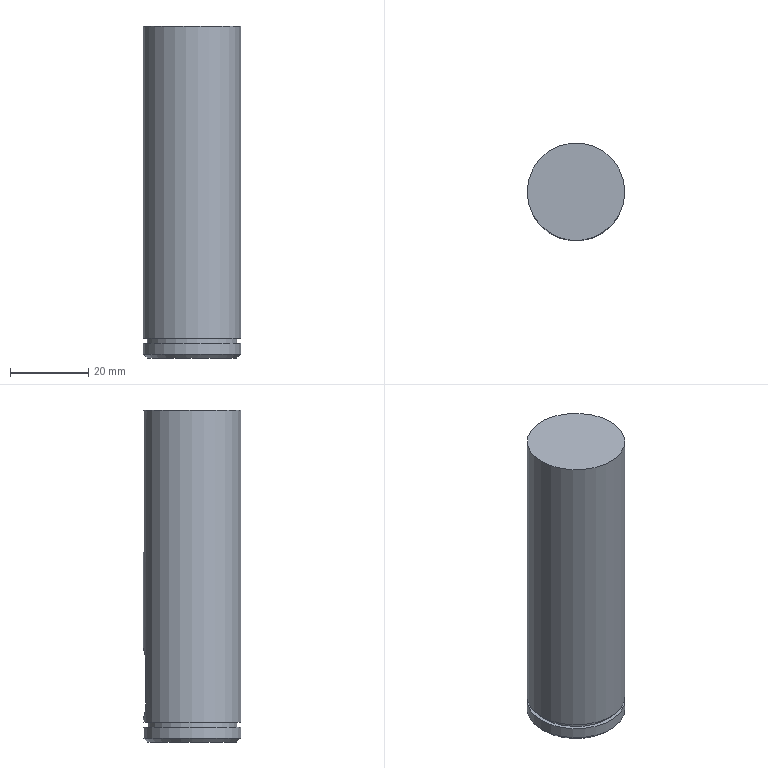Component | NX | MOTOR_SHAFT | 1 solid | 13 faces | box 25 x 25 x 85 mm | volume 41100 mm3 | plane 7 | cylinder 5 | cone 1 | commonest cylinder face diameters 25 x2 8 x2 23 x1
STEP:
#1=CARTESIAN_POINT('',(0.,0.,0.));
#2=DIRECTION('',(0.,0.,1.));
#3=DIRECTION('',(1.,0.,0.));
#4=AXIS2_PLACEMENT_3D('',#1,#2,#3);
#5=CARTESIAN_POINT('',(-610.675,308.181,-704.));
#6=VERTEX_POINT('',#5);
#7=CARTESIAN_POINT('',(-585.675,308.181,-704.));
#8=VERTEX_POINT('',#7);
#9=CARTESIAN_POINT('',(-598.175,308.181,-704.));
#10=DIRECTION('',(0.,0.,1.));
#11=DIRECTION('',(-1.,0.,0.));
#12=AXIS2_PLACEMENT_3D('',#9,#10,#11);
#13=CIRCLE('',#12,12.5);
#14=CARTESIAN_POINT('',(-598.175,308.181,-700.));
#15=DIRECTION('',(0.,0.,1.));
#16=DIRECTION('',(1.,0.,0.));
#17=AXIS2_PLACEMENT_3D('',#14,#15,#16);
#18=CYLINDRICAL_SURFACE('',#17,12.5);
#19=CARTESIAN_POINT('',(3.142,-4.));
#20=DIRECTION('',(1.,0.));
#21=VECTOR('',#20,1.);
#22=LINE('',#19,#21);
#23=(GEOMETRIC_REPRESENTATION_CONTEXT(2)PARAMETRIC_REPRESENTATION_CONTEXT()REPRESENTATION_CONTEXT('',''));
#24=DEFINITIONAL_REPRESENTATION('',(#22),#23);
#25=PCURVE('',#18,#24);
#26=CARTESIAN_POINT('',(-598.175,308.181,-704.));
#27=DIRECTION('',(0.,0.,1.));
#28=DIRECTION('',(1.,0.,0.));
#29=AXIS2_PLACEMENT_3D('',#26,#27,#28);
#30=CONICAL_SURFACE('',#29,12.5,0.7854);
#31=CARTESIAN_POINT('',(3.142,0.));
#32=DIRECTION('',(1.,0.));
#33=VECTOR('',#32,1.);
#34=LINE('',#31,#33);
#35=(GEOMETRIC_REPRESENTATION_CONTEXT(2)PARAMETRIC_REPRESENTATION_CONTEXT()REPRESENTATION_CONTEXT('',''));
#36=DEFINITIONAL_REPRESENTATION('',(#34),#35);
#37=PCURVE('',#30,#36);
#38=SURFACE_CURVE('',#13,(#25,#37),.PCURVE_S1.);
#39=EDGE_CURVE('',#6,#8,#38,.T.);
#40=ORIENTED_EDGE('',*,*,#39,.T.);
#41=CARTESIAN_POINT('',(-585.675,308.181,-701.2));
#42=VERTEX_POINT('',#41);
#43=CARTESIAN_POINT('',(-585.675,308.181,-704.));
#44=CARTESIAN_POINT('',(-585.675,308.181,-701.2));
#45=B_SPLINE_CURVE_WITH_KNOTS('',1,(#43,#44),.UNSPECIFIED.,.F.,.F.,(2,2),(-4.,-1.2),.PIECEWISE_BEZIER_KNOTS.);
#46=CARTESIAN_POINT('',(6.283,0.));
#47=DIRECTION('',(0.,1.));
#48=VECTOR('',#47,1.);
#49=LINE('',#46,#48);
#50=(GEOMETRIC_REPRESENTATION_CONTEXT(2)PARAMETRIC_REPRESENTATION_CONTEXT()REPRESENTATION_CONTEXT('',''));
#51=DEFINITIONAL_REPRESENTATION('',(#49),#50);
#52=PCURVE('',#18,#51);
#53=CARTESIAN_POINT('',(0.,0.));
#54=DIRECTION('',(0.,1.));
#55=VECTOR('',#54,1.);
#56=LINE('',#53,#55);
#57=(GEOMETRIC_REPRESENTATION_CONTEXT(2)PARAMETRIC_REPRESENTATION_CONTEXT()REPRESENTATION_CONTEXT('',''));
#58=DEFINITIONAL_REPRESENTATION('',(#56),#57);
#59=PCURVE('',#18,#58);
#60=SEAM_CURVE('',#45,(#52,#59),.PCURVE_S1.);
#61=EDGE_CURVE('',#8,#42,#60,.T.);
#62=ORIENTED_EDGE('',*,*,#61,.T.);
#63=CARTESIAN_POINT('',(-598.175,308.181,-701.2));
#64=DIRECTION('',(0.,0.,-1.));
#65=DIRECTION('',(1.,0.,0.));
#66=AXIS2_PLACEMENT_3D('',#63,#64,#65);
#67=CIRCLE('',#66,12.5);
#68=CARTESIAN_POINT('',(6.283,-1.2));
#69=DIRECTION('',(-1.,0.));
#70=VECTOR('',#69,1.);
#71=LINE('',#68,#70);
#72=(GEOMETRIC_REPRESENTATION_CONTEXT(2)PARAMETRIC_REPRESENTATION_CONTEXT()REPRESENTATION_CONTEXT('',''));
#73=DEFINITIONAL_REPRESENTATION('',(#71),#72);
#74=PCURVE('',#18,#73);
#75=CARTESIAN_POINT('',(-598.175,308.181,-701.2));
#76=DIRECTION('',(0.,0.,1.));
#77=DIRECTION('',(1.,0.,0.));
#78=AXIS2_PLACEMENT_3D('',#75,#76,#77);
#79=PLANE('',#78);
#80=CARTESIAN_POINT('',(12.5,0.));
#81=CARTESIAN_POINT('',(12.5,-21.651));
#82=CARTESIAN_POINT('',(-6.25,-10.825));
#83=CARTESIAN_POINT('',(-25.,-0.));
#84=CARTESIAN_POINT('',(-6.25,10.825));
#85=CARTESIAN_POINT('',(12.5,21.651));
#86=CARTESIAN_POINT('',(12.5,0.));
#87=(BOUNDED_CURVE()B_SPLINE_CURVE(2,(#80,#81,#82,#83,#84,#85,#86),.UNSPECIFIED.,.T.,.F.)B_SPLINE_CURVE_WITH_KNOTS((1,2,2,2,2,1),(-2.094,0.,2.094,4.189,6.283,8.378),.UNSPECIFIED.)CURVE()GEOMETRIC_REPRESENTATION_ITEM()RATIONAL_B_SPLINE_CURVE((1.,0.5,1.,0.5,1.,0.5,1.))REPRESENTATION_ITEM(''));
#88=(GEOMETRIC_REPRESENTATION_CONTEXT(2)PARAMETRIC_REPRESENTATION_CONTEXT()REPRESENTATION_CONTEXT('',''));
#89=DEFINITIONAL_REPRESENTATION('',(#87),#88);
#90=PCURVE('',#79,#89);
#91=SURFACE_CURVE('',#67,(#74,#90),.PCURVE_S1.);
#92=EDGE_CURVE('',#42,#42,#91,.T.);
#93=ORIENTED_EDGE('',*,*,#92,.T.);
#94=ORIENTED_EDGE('',*,*,#61,.F.);
#95=CARTESIAN_POINT('',(-598.175,308.181,-704.));
#96=DIRECTION('',(0.,0.,1.));
#97=DIRECTION('',(-1.,0.,0.));
#98=AXIS2_PLACEMENT_3D('',#95,#96,#97);
#99=CIRCLE('',#98,12.5);
#100=CARTESIAN_POINT('',(-3.142,-4.));
#101=DIRECTION('',(1.,0.));
#102=VECTOR('',#101,1.);
#103=LINE('',#100,#102);
#104=(GEOMETRIC_REPRESENTATION_CONTEXT(2)PARAMETRIC_REPRESENTATION_CONTEXT()REPRESENTATION_CONTEXT('',''));
#105=DEFINITIONAL_REPRESENTATION('',(#103),#104);
#106=PCURVE('',#18,#105);
#107=CARTESIAN_POINT('',(3.142,0.));
#108=DIRECTION('',(1.,0.));
#109=VECTOR('',#108,1.);
#110=LINE('',#107,#109);
#111=(GEOMETRIC_REPRESENTATION_CONTEXT(2)PARAMETRIC_REPRESENTATION_CONTEXT()REPRESENTATION_CONTEXT('',''));
#112=DEFINITIONAL_REPRESENTATION('',(#110),#111);
#113=PCURVE('',#30,#112);
#114=SURFACE_CURVE('',#99,(#106,#113),.PCURVE_S1.);
#115=EDGE_CURVE('',#8,#6,#114,.T.);
#116=ORIENTED_EDGE('',*,*,#115,.T.);
#117=EDGE_LOOP('',(#40,#62,#93,#94,#116));
#118=FACE_BOUND('',#117,.T.);
#119=ADVANCED_FACE('',(#118),#18,.T.);
#120=CARTESIAN_POINT('',(-609.675,308.181,-705.));
#121=VERTEX_POINT('',#120);
#122=CARTESIAN_POINT('',(-598.175,308.181,-705.));
#123=DIRECTION('',(0.,0.,-1.));
#124=DIRECTION('',(-1.,0.,0.));
#125=AXIS2_PLACEMENT_3D('',#122,#123,#124);
#126=CIRCLE('',#125,11.5);
#127=CARTESIAN_POINT('',(-598.175,308.181,-705.));
#128=DIRECTION('',(0.,0.,-1.));
#129=DIRECTION('',(-1.,0.,0.));
#130=AXIS2_PLACEMENT_3D('',#127,#128,#129);
#131=PLANE('',#130);
#132=CARTESIAN_POINT('',(0.,0.));
#133=DIRECTION('',(1.,0.));
#134=AXIS2_PLACEMENT_2D('',#132,#133);
#135=CIRCLE('',#134,11.5);
#136=(GEOMETRIC_REPRESENTATION_CONTEXT(2)PARAMETRIC_REPRESENTATION_CONTEXT()REPRESENTATION_CONTEXT('',''));
#137=DEFINITIONAL_REPRESENTATION('',(#135),#136);
#138=PCURVE('',#131,#137);
#139=CARTESIAN_POINT('',(9.425,-1.));
#140=DIRECTION('',(-1.,0.));
#141=VECTOR('',#140,1.);
#142=LINE('',#139,#141);
#143=(GEOMETRIC_REPRESENTATION_CONTEXT(2)PARAMETRIC_REPRESENTATION_CONTEXT()REPRESENTATION_CONTEXT('',''));
#144=DEFINITIONAL_REPRESENTATION('',(#142),#143);
#145=PCURVE('',#30,#144);
#146=SURFACE_CURVE('',#126,(#138,#145),.PCURVE_S1.);
#147=EDGE_CURVE('',#121,#121,#146,.T.);
#148=ORIENTED_EDGE('',*,*,#147,.T.);
#149=EDGE_LOOP('',(#148));
#150=FACE_BOUND('',#149,.T.);
#151=ADVANCED_FACE('',(#150),#131,.T.);
#152=ORIENTED_EDGE('',*,*,#147,.F.);
#153=CARTESIAN_POINT('',(-609.675,308.181,-705.));
#154=CARTESIAN_POINT('',(-610.675,308.181,-704.));
#155=B_SPLINE_CURVE_WITH_KNOTS('',1,(#153,#154),.UNSPECIFIED.,.F.,.F.,(2,2),(-1.414,0.),.PIECEWISE_BEZIER_KNOTS.);
#156=CARTESIAN_POINT('',(9.425,0.));
#157=DIRECTION('',(0.,1.));
#158=VECTOR('',#157,1.);
#159=LINE('',#156,#158);
#160=(GEOMETRIC_REPRESENTATION_CONTEXT(2)PARAMETRIC_REPRESENTATION_CONTEXT()REPRESENTATION_CONTEXT('',''));
#161=DEFINITIONAL_REPRESENTATION('',(#159),#160);
#162=PCURVE('',#30,#161);
#163=CARTESIAN_POINT('',(3.142,0.));
#164=DIRECTION('',(0.,1.));
#165=VECTOR('',#164,1.);
#166=LINE('',#163,#165);
#167=(GEOMETRIC_REPRESENTATION_CONTEXT(2)PARAMETRIC_REPRESENTATION_CONTEXT()REPRESENTATION_CONTEXT('',''));
#168=DEFINITIONAL_REPRESENTATION('',(#166),#167);
#169=PCURVE('',#30,#168);
#170=SEAM_CURVE('',#155,(#162,#169),.PCURVE_S1.);
#171=EDGE_CURVE('',#121,#6,#170,.T.);
#172=ORIENTED_EDGE('',*,*,#171,.T.);
#173=ORIENTED_EDGE('',*,*,#115,.F.);
#174=ORIENTED_EDGE('',*,*,#39,.F.);
#175=ORIENTED_EDGE('',*,*,#171,.F.);
#176=EDGE_LOOP('',(#152,#172,#173,#174,#175));
#177=FACE_BOUND('',#176,.T.);
#178=ADVANCED_FACE('',(#177),#30,.T.);
#179=CARTESIAN_POINT('',(-586.675,308.181,-700.));
#180=VERTEX_POINT('',#179);
#181=CARTESIAN_POINT('',(-598.175,308.181,-700.));
#182=DIRECTION('',(0.,0.,-1.));
#183=DIRECTION('',(1.,0.,0.));
#184=AXIS2_PLACEMENT_3D('',#181,#182,#183);
#185=CIRCLE('',#184,11.5);
#186=CARTESIAN_POINT('',(-598.175,308.181,-700.6));
#187=DIRECTION('',(0.,0.,1.));
#188=DIRECTION('',(1.,0.,0.));
#189=AXIS2_PLACEMENT_3D('',#186,#187,#188);
#190=CYLINDRICAL_SURFACE('',#189,11.5);
#191=CARTESIAN_POINT('',(6.283,0.6));
#192=DIRECTION('',(-1.,0.));
#193=VECTOR('',#192,1.);
#194=LINE('',#191,#193);
#195=(GEOMETRIC_REPRESENTATION_CONTEXT(2)PARAMETRIC_REPRESENTATION_CONTEXT()REPRESENTATION_CONTEXT('',''));
#196=DEFINITIONAL_REPRESENTATION('',(#194),#195);
#197=PCURVE('',#190,#196);
#198=CARTESIAN_POINT('',(-598.175,308.181,-700.));
#199=DIRECTION('',(0.,0.,1.));
#200=DIRECTION('',(1.,0.,0.));
#201=AXIS2_PLACEMENT_3D('',#198,#199,#200);
#202=PLANE('',#201);
#203=CARTESIAN_POINT('',(11.5,0.));
#204=CARTESIAN_POINT('',(11.5,-19.919));
#205=CARTESIAN_POINT('',(-5.75,-9.959));
#206=CARTESIAN_POINT('',(-23.,-0.));
#207=CARTESIAN_POINT('',(-5.75,9.959));
#208=CARTESIAN_POINT('',(11.5,19.919));
#209=CARTESIAN_POINT('',(11.5,0.));
#210=(BOUNDED_CURVE()B_SPLINE_CURVE(2,(#203,#204,#205,#206,#207,#208,#209),.UNSPECIFIED.,.T.,.F.)B_SPLINE_CURVE_WITH_KNOTS((1,2,2,2,2,1),(-2.094,0.,2.094,4.189,6.283,8.378),.UNSPECIFIED.)CURVE()GEOMETRIC_REPRESENTATION_ITEM()RATIONAL_B_SPLINE_CURVE((1.,0.5,1.,0.5,1.,0.5,1.))REPRESENTATION_ITEM(''));
#211=(GEOMETRIC_REPRESENTATION_CONTEXT(2)PARAMETRIC_REPRESENTATION_CONTEXT()REPRESENTATION_CONTEXT('',''));
#212=DEFINITIONAL_REPRESENTATION('',(#210),#211);
#213=PCURVE('',#202,#212);
#214=SURFACE_CURVE('',#185,(#197,#213),.PCURVE_S1.);
#215=EDGE_CURVE('',#180,#180,#214,.T.);
#216=ORIENTED_EDGE('',*,*,#215,.T.);
#217=CARTESIAN_POINT('',(-586.675,308.181,-701.2));
#218=VERTEX_POINT('',#217);
#219=CARTESIAN_POINT('',(-586.675,308.181,-701.2));
#220=CARTESIAN_POINT('',(-586.675,308.181,-700.));
#221=B_SPLINE_CURVE_WITH_KNOTS('',1,(#219,#220),.UNSPECIFIED.,.F.,.F.,(2,2),(-0.6,0.6),.PIECEWISE_BEZIER_KNOTS.);
#222=CARTESIAN_POINT('',(0.,0.));
#223=DIRECTION('',(0.,1.));
#224=VECTOR('',#223,1.);
#225=LINE('',#222,#224);
#226=(GEOMETRIC_REPRESENTATION_CONTEXT(2)PARAMETRIC_REPRESENTATION_CONTEXT()REPRESENTATION_CONTEXT('',''));
#227=DEFINITIONAL_REPRESENTATION('',(#225),#226);
#228=PCURVE('',#190,#227);
#229=CARTESIAN_POINT('',(6.283,0.));
#230=DIRECTION('',(0.,1.));
#231=VECTOR('',#230,1.);
#232=LINE('',#229,#231);
#233=(GEOMETRIC_REPRESENTATION_CONTEXT(2)PARAMETRIC_REPRESENTATION_CONTEXT()REPRESENTATION_CONTEXT('',''));
#234=DEFINITIONAL_REPRESENTATION('',(#232),#233);
#235=PCURVE('',#190,#234);
#236=SEAM_CURVE('',#221,(#228,#235),.PCURVE_S1.);
#237=EDGE_CURVE('',#218,#180,#236,.T.);
#238=ORIENTED_EDGE('',*,*,#237,.F.);
#239=CARTESIAN_POINT('',(-598.175,308.181,-701.2));
#240=DIRECTION('',(0.,0.,-1.));
#241=DIRECTION('',(1.,0.,0.));
#242=AXIS2_PLACEMENT_3D('',#239,#240,#241);
#243=CIRCLE('',#242,11.5);
#244=CARTESIAN_POINT('',(6.283,-0.6));
#245=DIRECTION('',(-1.,0.));
#246=VECTOR('',#245,1.);
#247=LINE('',#244,#246);
#248=(GEOMETRIC_REPRESENTATION_CONTEXT(2)PARAMETRIC_REPRESENTATION_CONTEXT()REPRESENTATION_CONTEXT('',''));
#249=DEFINITIONAL_REPRESENTATION('',(#247),#248);
#250=PCURVE('',#190,#249);
#251=CARTESIAN_POINT('',(11.5,0.));
#252=CARTESIAN_POINT('',(11.5,-19.919));
#253=CARTESIAN_POINT('',(-5.75,-9.959));
#254=CARTESIAN_POINT('',(-23.,-0.));
#255=CARTESIAN_POINT('',(-5.75,9.959));
#256=CARTESIAN_POINT('',(11.5,19.919));
#257=CARTESIAN_POINT('',(11.5,0.));
#258=(BOUNDED_CURVE()B_SPLINE_CURVE(2,(#251,#252,#253,#254,#255,#256,#257),.UNSPECIFIED.,.T.,.F.)B_SPLINE_CURVE_WITH_KNOTS((1,2,2,2,2,1),(-2.094,0.,2.094,4.189,6.283,8.378),.UNSPECIFIED.)CURVE()GEOMETRIC_REPRESENTATION_ITEM()RATIONAL_B_SPLINE_CURVE((1.,0.5,1.,0.5,1.,0.5,1.))REPRESENTATION_ITEM(''));
#259=(GEOMETRIC_REPRESENTATION_CONTEXT(2)PARAMETRIC_REPRESENTATION_CONTEXT()REPRESENTATION_CONTEXT('',''));
#260=DEFINITIONAL_REPRESENTATION('',(#258),#259);
#261=PCURVE('',#79,#260);
#262=SURFACE_CURVE('',#243,(#250,#261),.PCURVE_S1.);
#263=EDGE_CURVE('',#218,#218,#262,.T.);
#264=ORIENTED_EDGE('',*,*,#263,.F.);
#265=ORIENTED_EDGE('',*,*,#237,.T.);
#266=EDGE_LOOP('',(#216,#238,#264,#265));
#267=FACE_BOUND('',#266,.T.);
#268=ADVANCED_FACE('',(#267),#190,.T.);
#269=ORIENTED_EDGE('',*,*,#92,.F.);
#270=EDGE_LOOP('',(#269));
#271=FACE_BOUND('',#270,.T.);
#272=ORIENTED_EDGE('',*,*,#263,.T.);
#273=EDGE_LOOP('',(#272));
#274=FACE_BOUND('',#273,.T.);
#275=ADVANCED_FACE('',(#271,#274),#79,.T.);
#276=CARTESIAN_POINT('',(-585.675,308.181,-700.));
#277=VERTEX_POINT('',#276);
#278=CARTESIAN_POINT('',(-598.175,308.181,-700.));
#279=DIRECTION('',(0.,0.,-1.));
#280=DIRECTION('',(1.,0.,0.));
#281=AXIS2_PLACEMENT_3D('',#278,#279,#280);
#282=CIRCLE('',#281,12.5);
#283=CARTESIAN_POINT('',(12.5,0.));
#284=CARTESIAN_POINT('',(12.5,-21.651));
#285=CARTESIAN_POINT('',(-6.25,-10.825));
#286=CARTESIAN_POINT('',(-25.,-0.));
#287=CARTESIAN_POINT('',(-6.25,10.825));
#288=CARTESIAN_POINT('',(12.5,21.651));
#289=CARTESIAN_POINT('',(12.5,0.));
#290=(BOUNDED_CURVE()B_SPLINE_CURVE(2,(#283,#284,#285,#286,#287,#288,#289),.UNSPECIFIED.,.T.,.F.)B_SPLINE_CURVE_WITH_KNOTS((1,2,2,2,2,1),(-2.094,0.,2.094,4.189,6.283,8.378),.UNSPECIFIED.)CURVE()GEOMETRIC_REPRESENTATION_ITEM()RATIONAL_B_SPLINE_CURVE((1.,0.5,1.,0.5,1.,0.5,1.))REPRESENTATION_ITEM(''));
#291=(GEOMETRIC_REPRESENTATION_CONTEXT(2)PARAMETRIC_REPRESENTATION_CONTEXT()REPRESENTATION_CONTEXT('',''));
#292=DEFINITIONAL_REPRESENTATION('',(#290),#291);
#293=PCURVE('',#202,#292);
#294=CARTESIAN_POINT('',(-598.175,308.181,-700.));
#295=DIRECTION('',(0.,0.,1.));
#296=DIRECTION('',(1.,0.,0.));
#297=AXIS2_PLACEMENT_3D('',#294,#295,#296);
#298=CYLINDRICAL_SURFACE('',#297,12.5);
#299=CARTESIAN_POINT('',(6.283,0.));
#300=DIRECTION('',(-1.,0.));
#301=VECTOR('',#300,1.);
#302=LINE('',#299,#301);
#303=(GEOMETRIC_REPRESENTATION_CONTEXT(2)PARAMETRIC_REPRESENTATION_CONTEXT()REPRESENTATION_CONTEXT('',''));
#304=DEFINITIONAL_REPRESENTATION('',(#302),#303);
#305=PCURVE('',#298,#304);
#306=SURFACE_CURVE('',#282,(#293,#305),.PCURVE_S1.);
#307=EDGE_CURVE('',#277,#277,#306,.T.);
#308=ORIENTED_EDGE('',*,*,#307,.T.);
#309=EDGE_LOOP('',(#308));
#310=FACE_BOUND('',#309,.T.);
#311=ORIENTED_EDGE('',*,*,#215,.F.);
#312=EDGE_LOOP('',(#311));
#313=FACE_BOUND('',#312,.T.);
#314=ADVANCED_FACE('',(#310,#313),#202,.F.);
#315=CARTESIAN_POINT('',(-594.175,316.681,-695.));
#316=VERTEX_POINT('',#315);
#317=CARTESIAN_POINT('',(-594.175,316.681,-685.));
#318=VERTEX_POINT('',#317);
#319=CARTESIAN_POINT('',(-594.175,316.681,-681.));
#320=DIRECTION('',(0.,-0.,1.));
#321=VECTOR('',#320,1.);
#322=LINE('',#319,#321);
#323=CARTESIAN_POINT('',(-594.175,316.681,-681.));
#324=DIRECTION('',(0.,1.,0.));
#325=DIRECTION('',(0.,-0.,1.));
#326=AXIS2_PLACEMENT_3D('',#323,#324,#325);
#327=PLANE('',#326);
#328=CARTESIAN_POINT('',(0.,0.));
#329=DIRECTION('',(1.,0.));
#330=VECTOR('',#329,1.);
#331=LINE('',#328,#330);
#332=(GEOMETRIC_REPRESENTATION_CONTEXT(2)PARAMETRIC_REPRESENTATION_CONTEXT()REPRESENTATION_CONTEXT('',''));
#333=DEFINITIONAL_REPRESENTATION('',(#331),#332);
#334=PCURVE('',#327,#333);
#335=CARTESIAN_POINT('',(-594.175,308.181,-700.));
#336=DIRECTION('',(1.,0.,0.));
#337=DIRECTION('',(0.,0.,-1.));
#338=AXIS2_PLACEMENT_3D('',#335,#336,#337);
#339=PLANE('',#338);
#340=CARTESIAN_POINT('',(-19.,8.5));
#341=DIRECTION('',(-1.,-0.));
#342=VECTOR('',#341,1.);
#343=LINE('',#340,#342);
#344=(GEOMETRIC_REPRESENTATION_CONTEXT(2)PARAMETRIC_REPRESENTATION_CONTEXT()REPRESENTATION_CONTEXT('',''));
#345=DEFINITIONAL_REPRESENTATION('',(#343),#344);
#346=PCURVE('',#339,#345);
#347=SURFACE_CURVE('',#322,(#334,#346),.PCURVE_S1.);
#348=EDGE_CURVE('',#316,#318,#347,.T.);
#349=ORIENTED_EDGE('',*,*,#348,.F.);
#350=CARTESIAN_POINT('',(-602.175,316.681,-695.));
#351=VERTEX_POINT('',#350);
#352=CARTESIAN_POINT('',(-598.175,316.681,-695.));
#353=DIRECTION('',(0.,1.,0.));
#354=DIRECTION('',(0.,-0.,1.));
#355=AXIS2_PLACEMENT_3D('',#352,#353,#354);
#356=CIRCLE('',#355,4.);
#357=CARTESIAN_POINT('',(-14.,-4.));
#358=DIRECTION('',(1.,0.));
#359=AXIS2_PLACEMENT_2D('',#357,#358);
#360=CIRCLE('',#359,4.);
#361=(GEOMETRIC_REPRESENTATION_CONTEXT(2)PARAMETRIC_REPRESENTATION_CONTEXT()REPRESENTATION_CONTEXT('',''));
#362=DEFINITIONAL_REPRESENTATION('',(#360),#361);
#363=PCURVE('',#327,#362);
#364=CARTESIAN_POINT('',(-598.175,316.681,-695.));
#365=DIRECTION('',(0.,1.,0.));
#366=DIRECTION('',(0.,-0.,1.));
#367=AXIS2_PLACEMENT_3D('',#364,#365,#366);
#368=CYLINDRICAL_SURFACE('',#367,4.);
#369=CARTESIAN_POINT('',(0.,0.));
#370=DIRECTION('',(1.,0.));
#371=VECTOR('',#370,1.);
#372=LINE('',#369,#371);
#373=(GEOMETRIC_REPRESENTATION_CONTEXT(2)PARAMETRIC_REPRESENTATION_CONTEXT()REPRESENTATION_CONTEXT('',''));
#374=DEFINITIONAL_REPRESENTATION('',(#372),#373);
#375=PCURVE('',#368,#374);
#376=SURFACE_CURVE('',#356,(#363,#375),.PCURVE_S1.);
#377=EDGE_CURVE('',#316,#351,#376,.T.);
#378=ORIENTED_EDGE('',*,*,#377,.T.);
#379=CARTESIAN_POINT('',(-602.175,316.681,-685.));
#380=VERTEX_POINT('',#379);
#381=CARTESIAN_POINT('',(-602.175,316.681,-681.));
#382=DIRECTION('',(0.,-0.,1.));
#383=VECTOR('',#382,1.);
#384=LINE('',#381,#383);
#385=CARTESIAN_POINT('',(0.,-8.));
#386=DIRECTION('',(1.,0.));
#387=VECTOR('',#386,1.);
#388=LINE('',#385,#387);
#389=(GEOMETRIC_REPRESENTATION_CONTEXT(2)PARAMETRIC_REPRESENTATION_CONTEXT()REPRESENTATION_CONTEXT('',''));
#390=DEFINITIONAL_REPRESENTATION('',(#388),#389);
#391=PCURVE('',#327,#390);
#392=CARTESIAN_POINT('',(-602.175,308.181,-700.));
#393=DIRECTION('',(1.,0.,0.));
#394=DIRECTION('',(0.,0.,-1.));
#395=AXIS2_PLACEMENT_3D('',#392,#393,#394);
#396=PLANE('',#395);
#397=CARTESIAN_POINT('',(-19.,8.5));
#398=DIRECTION('',(-1.,-0.));
#399=VECTOR('',#398,1.);
#400=LINE('',#397,#399);
#401=(GEOMETRIC_REPRESENTATION_CONTEXT(2)PARAMETRIC_REPRESENTATION_CONTEXT()REPRESENTATION_CONTEXT('',''));
#402=DEFINITIONAL_REPRESENTATION('',(#400),#401);
#403=PCURVE('',#396,#402);
#404=SURFACE_CURVE('',#384,(#391,#403),.PCURVE_S1.);
#405=EDGE_CURVE('',#351,#380,#404,.T.);
#406=ORIENTED_EDGE('',*,*,#405,.T.);
#407=CARTESIAN_POINT('',(-598.175,316.681,-685.));
#408=DIRECTION('',(0.,1.,0.));
#409=DIRECTION('',(0.,-0.,1.));
#410=AXIS2_PLACEMENT_3D('',#407,#408,#409);
#411=CIRCLE('',#410,4.);
#412=CARTESIAN_POINT('',(-4.,-4.));
#413=DIRECTION('',(1.,0.));
#414=AXIS2_PLACEMENT_2D('',#412,#413);
#415=CIRCLE('',#414,4.);
#416=(GEOMETRIC_REPRESENTATION_CONTEXT(2)PARAMETRIC_REPRESENTATION_CONTEXT()REPRESENTATION_CONTEXT('',''));
#417=DEFINITIONAL_REPRESENTATION('',(#415),#416);
#418=PCURVE('',#327,#417);
#419=CARTESIAN_POINT('',(-598.175,308.181,-685.));
#420=DIRECTION('',(0.,1.,0.));
#421=DIRECTION('',(0.,0.,1.));
#422=AXIS2_PLACEMENT_3D('',#419,#420,#421);
#423=CYLINDRICAL_SURFACE('',#422,4.);
#424=CARTESIAN_POINT('',(-6.283,8.5));
#425=DIRECTION('',(1.,0.));
#426=VECTOR('',#425,1.);
#427=LINE('',#424,#426);
#428=(GEOMETRIC_REPRESENTATION_CONTEXT(2)PARAMETRIC_REPRESENTATION_CONTEXT()REPRESENTATION_CONTEXT('',''));
#429=DEFINITIONAL_REPRESENTATION('',(#427),#428);
#430=PCURVE('',#423,#429);
#431=SURFACE_CURVE('',#411,(#418,#430),.PCURVE_S1.);
#432=EDGE_CURVE('',#380,#318,#431,.T.);
#433=ORIENTED_EDGE('',*,*,#432,.T.);
#434=EDGE_LOOP('',(#349,#378,#406,#433));
#435=FACE_BOUND('',#434,.T.);
#436=ADVANCED_FACE('',(#435),#327,.T.);
#437=CARTESIAN_POINT('',(-585.675,308.181,-620.));
#438=VERTEX_POINT('',#437);
#439=CARTESIAN_POINT('',(-598.175,308.181,-620.));
#440=DIRECTION('',(0.,0.,-1.));
#441=DIRECTION('',(1.,0.,0.));
#442=AXIS2_PLACEMENT_3D('',#439,#440,#441);
#443=CIRCLE('',#442,12.5);
#444=CARTESIAN_POINT('',(-598.175,308.181,-620.));
#445=DIRECTION('',(0.,0.,1.));
#446=DIRECTION('',(1.,0.,0.));
#447=AXIS2_PLACEMENT_3D('',#444,#445,#446);
#448=PLANE('',#447);
#449=CARTESIAN_POINT('',(12.5,0.));
#450=CARTESIAN_POINT('',(12.5,-21.651));
#451=CARTESIAN_POINT('',(-6.25,-10.825));
#452=CARTESIAN_POINT('',(-25.,-0.));
#453=CARTESIAN_POINT('',(-6.25,10.825));
#454=CARTESIAN_POINT('',(12.5,21.651));
#455=CARTESIAN_POINT('',(12.5,0.));
#456=(BOUNDED_CURVE()B_SPLINE_CURVE(2,(#449,#450,#451,#452,#453,#454,#455),.UNSPECIFIED.,.T.,.F.)B_SPLINE_CURVE_WITH_KNOTS((1,2,2,2,2,1),(-2.094,0.,2.094,4.189,6.283,8.378),.UNSPECIFIED.)CURVE()GEOMETRIC_REPRESENTATION_ITEM()RATIONAL_B_SPLINE_CURVE((1.,0.5,1.,0.5,1.,0.5,1.))REPRESENTATION_ITEM(''));
#457=(GEOMETRIC_REPRESENTATION_CONTEXT(2)PARAMETRIC_REPRESENTATION_CONTEXT()REPRESENTATION_CONTEXT('',''));
#458=DEFINITIONAL_REPRESENTATION('',(#456),#457);
#459=PCURVE('',#448,#458);
#460=CARTESIAN_POINT('',(6.283,80.));
#461=DIRECTION('',(-1.,0.));
#462=VECTOR('',#461,1.);
#463=LINE('',#460,#462);
#464=(GEOMETRIC_REPRESENTATION_CONTEXT(2)PARAMETRIC_REPRESENTATION_CONTEXT()REPRESENTATION_CONTEXT('',''));
#465=DEFINITIONAL_REPRESENTATION('',(#463),#464);
#466=PCURVE('',#298,#465);
#467=SURFACE_CURVE('',#443,(#459,#466),.PCURVE_S1.);
#468=EDGE_CURVE('',#438,#438,#467,.T.);
#469=ORIENTED_EDGE('',*,*,#468,.F.);
#470=EDGE_LOOP('',(#469));
#471=FACE_BOUND('',#470,.T.);
#472=ADVANCED_FACE('',(#471),#448,.T.);
#473=CARTESIAN_POINT('',(-602.175,320.024,-695.));
#474=VERTEX_POINT('',#473);
#475=CARTESIAN_POINT('',(-602.175,320.024,-695.));
#476=DIRECTION('',(0.,1.,0.));
#477=VECTOR('',#476,1.);
#478=LINE('',#475,#477);
#479=CARTESIAN_POINT('',(4.712,3.343));
#480=DIRECTION('',(0.,1.));
#481=VECTOR('',#480,1.);
#482=LINE('',#479,#481);
#483=(GEOMETRIC_REPRESENTATION_CONTEXT(2)PARAMETRIC_REPRESENTATION_CONTEXT()REPRESENTATION_CONTEXT('',''));
#484=DEFINITIONAL_REPRESENTATION('',(#482),#483);
#485=PCURVE('',#368,#484);
#486=CARTESIAN_POINT('',(-5.,11.843));
#487=DIRECTION('',(-0.,1.));
#488=VECTOR('',#487,1.);
#489=LINE('',#486,#488);
#490=(GEOMETRIC_REPRESENTATION_CONTEXT(2)PARAMETRIC_REPRESENTATION_CONTEXT()REPRESENTATION_CONTEXT('',''));
#491=DEFINITIONAL_REPRESENTATION('',(#489),#490);
#492=PCURVE('',#396,#491);
#493=SURFACE_CURVE('',#478,(#485,#492),.PCURVE_S1.);
#494=EDGE_CURVE('',#351,#474,#493,.T.);
#495=ORIENTED_EDGE('',*,*,#494,.T.);
#496=CARTESIAN_POINT('',(-594.175,320.024,-695.));
#497=VERTEX_POINT('',#496);
#498=CARTESIAN_POINT('',(-602.175,320.024,-695.));
#499=CARTESIAN_POINT('',(-602.175,320.024,-695.435));
#500=CARTESIAN_POINT('',(-602.102,320.049,-695.875));
#501=CARTESIAN_POINT('',(-601.963,320.094,-696.285));
#502=CARTESIAN_POINT('',(-601.824,320.138,-696.694));
#503=CARTESIAN_POINT('',(-601.617,320.201,-697.083));
#504=CARTESIAN_POINT('',(-601.357,320.27,-697.424));
#505=CARTESIAN_POINT('',(-601.088,320.34,-697.777));
#506=CARTESIAN_POINT('',(-600.757,320.418,-698.087));
#507=CARTESIAN_POINT('',(-600.388,320.484,-698.332));
#508=CARTESIAN_POINT('',(-600.01,320.552,-698.583));
#509=CARTESIAN_POINT('',(-599.58,320.61,-698.773));
#510=CARTESIAN_POINT('',(-599.136,320.644,-698.883));
#511=CARTESIAN_POINT('',(-598.823,320.668,-698.96));
#512=CARTESIAN_POINT('',(-598.498,320.681,-699.));
#513=CARTESIAN_POINT('',(-598.175,320.681,-699.));
#514=CARTESIAN_POINT('',(-597.74,320.681,-699.));
#515=CARTESIAN_POINT('',(-597.299,320.657,-698.927));
#516=CARTESIAN_POINT('',(-596.888,320.615,-698.787));
#517=CARTESIAN_POINT('',(-596.478,320.573,-698.648));
#518=CARTESIAN_POINT('',(-596.088,320.511,-698.439));
#519=CARTESIAN_POINT('',(-595.747,320.443,-698.179));
#520=CARTESIAN_POINT('',(-595.396,320.374,-697.91));
#521=CARTESIAN_POINT('',(-595.086,320.296,-697.579));
#522=CARTESIAN_POINT('',(-594.842,320.229,-697.21));
#523=CARTESIAN_POINT('',(-594.591,320.159,-696.832));
#524=CARTESIAN_POINT('',(-594.402,320.099,-696.403));
#525=CARTESIAN_POINT('',(-594.292,320.063,-695.959));
#526=CARTESIAN_POINT('',(-594.215,320.038,-695.647));
#527=CARTESIAN_POINT('',(-594.175,320.024,-695.322));
#528=CARTESIAN_POINT('',(-594.175,320.024,-695.));
#529=B_SPLINE_CURVE_WITH_KNOTS('',3,(#498,#499,#500,#501,#502,#503,#504,#505,#506,#507,#508,#509,#510,#511,#512,#513,#514,#515,#516,#517,#518,#519,#520,#521,#522,#523,#524,#525,#526,#527,#528),.UNSPECIFIED.,.F.,.F.,(4,3,3,3,3,3,3,3,3,3,4),(0.,0.1037,0.2071,0.314,0.4235,0.5,0.6038,0.7074,0.8141,0.9237,1.),.UNSPECIFIED.);
#530=CARTESIAN_POINT('',(4.712,3.343));
#531=CARTESIAN_POINT('',(4.689,3.343));
#532=CARTESIAN_POINT('',(4.641,3.345));
#533=CARTESIAN_POINT('',(4.569,3.356));
#534=CARTESIAN_POINT('',(4.497,3.373));
#535=CARTESIAN_POINT('',(4.425,3.396));
#536=CARTESIAN_POINT('',(4.354,3.425));
#537=CARTESIAN_POINT('',(4.283,3.459));
#538=CARTESIAN_POINT('',(4.211,3.497));
#539=CARTESIAN_POINT('',(4.14,3.539));
#540=CARTESIAN_POINT('',(4.069,3.583));
#541=CARTESIAN_POINT('',(3.999,3.629));
#542=CARTESIAN_POINT('',(3.928,3.675));
#543=CARTESIAN_POINT('',(3.856,3.722));
#544=CARTESIAN_POINT('',(3.785,3.768));
#545=CARTESIAN_POINT('',(3.715,3.811));
#546=CARTESIAN_POINT('',(3.644,3.851));
#547=CARTESIAN_POINT('',(3.572,3.888));
#548=CARTESIAN_POINT('',(3.501,3.921));
#549=CARTESIAN_POINT('',(3.429,3.949));
#550=CARTESIAN_POINT('',(3.358,3.971));
#551=CARTESIAN_POINT('',(3.286,3.988));
#552=CARTESIAN_POINT('',(3.214,3.998));
#553=CARTESIAN_POINT('',(3.141,4.001));
#554=CARTESIAN_POINT('',(3.07,3.998));
#555=CARTESIAN_POINT('',(2.998,3.988));
#556=CARTESIAN_POINT('',(2.926,3.972));
#557=CARTESIAN_POINT('',(2.854,3.949));
#558=CARTESIAN_POINT('',(2.783,3.922));
#559=CARTESIAN_POINT('',(2.712,3.889));
#560=CARTESIAN_POINT('',(2.64,3.852));
#561=CARTESIAN_POINT('',(2.569,3.811));
#562=CARTESIAN_POINT('',(2.498,3.768));
#563=CARTESIAN_POINT('',(2.428,3.723));
#564=CARTESIAN_POINT('',(2.357,3.676));
#565=CARTESIAN_POINT('',(2.285,3.629));
#566=CARTESIAN_POINT('',(2.214,3.583));
#567=CARTESIAN_POINT('',(2.144,3.539));
#568=CARTESIAN_POINT('',(2.073,3.498));
#569=CARTESIAN_POINT('',(2.001,3.459));
#570=CARTESIAN_POINT('',(1.93,3.425));
#571=CARTESIAN_POINT('',(1.859,3.396));
#572=CARTESIAN_POINT('',(1.787,3.373));
#573=CARTESIAN_POINT('',(1.715,3.356));
#574=CARTESIAN_POINT('',(1.643,3.345));
#575=CARTESIAN_POINT('',(1.595,3.343));
#576=CARTESIAN_POINT('',(1.571,3.343));
#577=B_SPLINE_CURVE_WITH_KNOTS('',3,(#530,#531,#532,#533,#534,#535,#536,#537,#538,#539,#540,#541,#542,#543,#544,#545,#546,#547,#548,#549,#550,#551,#552,#553,#554,#555,#556,#557,#558,#559,#560,#561,#562,#563,#564,#565,#566,#567,#568,#569,#570,#571,#572,#573,#574,#575,#576),.UNSPECIFIED.,.F.,.F.,(4,1,1,1,1,1,1,1,1,1,1,1,1,1,1,1,1,1,1,1,1,1,1,1,1,1,1,1,1,1,1,1,1,1,1,1,1,1,1,1,1,1,1,1,4),(0.,0.02273,0.04545,0.06818,0.09091,0.1136,0.1364,0.1591,0.1818,0.2045,0.2273,0.25,0.2727,0.2955,0.3182,0.3409,0.3636,0.3864,0.4091,0.4318,0.4545,0.4773,0.5,0.5227,0.5455,0.5682,0.5909,0.6136,0.6364,0.6591,0.6818,0.7045,0.7273,0.75,0.7727,0.7955,0.8182,0.8409,0.8636,0.8864,0.9091,0.9318,0.9545,0.9773,1.),.QUASI_UNIFORM_KNOTS.);
#578=(GEOMETRIC_REPRESENTATION_CONTEXT(2)PARAMETRIC_REPRESENTATION_CONTEXT()REPRESENTATION_CONTEXT('',''));
#579=DEFINITIONAL_REPRESENTATION('',(#577),#578);
#580=PCURVE('',#368,#579);
#581=CARTESIAN_POINT('',(1.897,5.));
#582=CARTESIAN_POINT('',(1.897,4.905));
#583=CARTESIAN_POINT('',(1.896,4.714));
#584=CARTESIAN_POINT('',(1.893,4.427));
#585=CARTESIAN_POINT('',(1.889,4.144));
#586=CARTESIAN_POINT('',(1.883,3.866));
#587=CARTESIAN_POINT('',(1.875,3.596));
#588=CARTESIAN_POINT('',(1.866,3.333));
#589=CARTESIAN_POINT('',(1.856,3.077));
#590=CARTESIAN_POINT('',(1.843,2.832));
#591=CARTESIAN_POINT('',(1.83,2.599));
#592=CARTESIAN_POINT('',(1.815,2.379));
#593=CARTESIAN_POINT('',(1.799,2.171));
#594=CARTESIAN_POINT('',(1.782,1.977));
#595=CARTESIAN_POINT('',(1.764,1.798));
#596=CARTESIAN_POINT('',(1.745,1.636));
#597=CARTESIAN_POINT('',(1.726,1.491));
#598=CARTESIAN_POINT('',(1.705,1.363));
#599=CARTESIAN_POINT('',(1.684,1.253));
#600=CARTESIAN_POINT('',(1.662,1.161));
#601=CARTESIAN_POINT('',(1.64,1.09));
#602=CARTESIAN_POINT('',(1.617,1.038));
#603=CARTESIAN_POINT('',(1.594,1.007));
#604=CARTESIAN_POINT('',(1.571,0.9965));
#605=CARTESIAN_POINT('',(1.548,1.007));
#606=CARTESIAN_POINT('',(1.525,1.038));
#607=CARTESIAN_POINT('',(1.502,1.09));
#608=CARTESIAN_POINT('',(1.48,1.161));
#609=CARTESIAN_POINT('',(1.458,1.251));
#610=CARTESIAN_POINT('',(1.437,1.361));
#611=CARTESIAN_POINT('',(1.416,1.489));
#612=CARTESIAN_POINT('',(1.396,1.635));
#613=CARTESIAN_POINT('',(1.377,1.797));
#614=CARTESIAN_POINT('',(1.359,1.975));
#615=CARTESIAN_POINT('',(1.342,2.169));
#616=CARTESIAN_POINT('',(1.326,2.377));
#617=CARTESIAN_POINT('',(1.312,2.598));
#618=CARTESIAN_POINT('',(1.298,2.83));
#619=CARTESIAN_POINT('',(1.286,3.074));
#620=CARTESIAN_POINT('',(1.276,3.329));
#621=CARTESIAN_POINT('',(1.266,3.593));
#622=CARTESIAN_POINT('',(1.259,3.864));
#623=CARTESIAN_POINT('',(1.253,4.14));
#624=CARTESIAN_POINT('',(1.248,4.424));
#625=CARTESIAN_POINT('',(1.246,4.712));
#626=CARTESIAN_POINT('',(1.245,4.904));
#627=CARTESIAN_POINT('',(1.245,5.));
#628=B_SPLINE_CURVE_WITH_KNOTS('',3,(#581,#582,#583,#584,#585,#586,#587,#588,#589,#590,#591,#592,#593,#594,#595,#596,#597,#598,#599,#600,#601,#602,#603,#604,#605,#606,#607,#608,#609,#610,#611,#612,#613,#614,#615,#616,#617,#618,#619,#620,#621,#622,#623,#624,#625,#626,#627),.UNSPECIFIED.,.F.,.F.,(4,1,1,1,1,1,1,1,1,1,1,1,1,1,1,1,1,1,1,1,1,1,1,1,1,1,1,1,1,1,1,1,1,1,1,1,1,1,1,1,1,1,1,1,4),(0.,0.02273,0.04545,0.06818,0.09091,0.1136,0.1364,0.1591,0.1818,0.2045,0.2273,0.25,0.2727,0.2955,0.3182,0.3409,0.3636,0.3864,0.4091,0.4318,0.4545,0.4773,0.5,0.5227,0.5455,0.5682,0.5909,0.6136,0.6364,0.6591,0.6818,0.7045,0.7273,0.75,0.7727,0.7955,0.8182,0.8409,0.8636,0.8864,0.9091,0.9318,0.9545,0.9773,1.),.QUASI_UNIFORM_KNOTS.);
#629=(GEOMETRIC_REPRESENTATION_CONTEXT(2)PARAMETRIC_REPRESENTATION_CONTEXT()REPRESENTATION_CONTEXT('',''));
#630=DEFINITIONAL_REPRESENTATION('',(#628),#629);
#631=PCURVE('',#298,#630);
#632=SURFACE_CURVE('',#529,(#580,#631),.PCURVE_S1.);
#633=EDGE_CURVE('',#474,#497,#632,.T.);
#634=ORIENTED_EDGE('',*,*,#633,.T.);
#635=CARTESIAN_POINT('',(-594.175,308.181,-695.));
#636=DIRECTION('',(0.,-1.,-0.));
#637=VECTOR('',#636,1.);
#638=LINE('',#635,#637);
#639=CARTESIAN_POINT('',(1.571,-8.5));
#640=DIRECTION('',(0.,-1.));
#641=VECTOR('',#640,1.);
#642=LINE('',#639,#641);
#643=(GEOMETRIC_REPRESENTATION_CONTEXT(2)PARAMETRIC_REPRESENTATION_CONTEXT()REPRESENTATION_CONTEXT('',''));
#644=DEFINITIONAL_REPRESENTATION('',(#642),#643);
#645=PCURVE('',#368,#644);
#646=CARTESIAN_POINT('',(-5.,0.));
#647=DIRECTION('',(0.,-1.));
#648=VECTOR('',#647,1.);
#649=LINE('',#646,#648);
#650=(GEOMETRIC_REPRESENTATION_CONTEXT(2)PARAMETRIC_REPRESENTATION_CONTEXT()REPRESENTATION_CONTEXT('',''));
#651=DEFINITIONAL_REPRESENTATION('',(#649),#650);
#652=PCURVE('',#339,#651);
#653=SURFACE_CURVE('',#638,(#645,#652),.PCURVE_S1.);
#654=EDGE_CURVE('',#497,#316,#653,.T.);
#655=ORIENTED_EDGE('',*,*,#654,.T.);
#656=ORIENTED_EDGE('',*,*,#377,.T.);
#657=EDGE_LOOP('',(#495,#634,#655,#656));
#658=FACE_BOUND('',#657,.F.);
#659=ADVANCED_FACE('',(#658),#368,.F.);
#660=ORIENTED_EDGE('',*,*,#405,.F.);
#661=ORIENTED_EDGE('',*,*,#494,.T.);
#662=CARTESIAN_POINT('',(-602.175,320.024,-685.));
#663=VERTEX_POINT('',#662);
#664=CARTESIAN_POINT('',(-602.175,320.024,-700.));
#665=DIRECTION('',(0.,0.,-1.));
#666=VECTOR('',#665,1.);
#667=LINE('',#664,#666);
#668=CARTESIAN_POINT('',(0.,11.843));
#669=DIRECTION('',(1.,0.));
#670=VECTOR('',#669,1.);
#671=LINE('',#668,#670);
#672=(GEOMETRIC_REPRESENTATION_CONTEXT(2)PARAMETRIC_REPRESENTATION_CONTEXT()REPRESENTATION_CONTEXT('',''));
#673=DEFINITIONAL_REPRESENTATION('',(#671),#672);
#674=PCURVE('',#396,#673);
#675=CARTESIAN_POINT('',(1.897,0.));
#676=DIRECTION('',(0.,-1.));
#677=VECTOR('',#676,1.);
#678=LINE('',#675,#677);
#679=(GEOMETRIC_REPRESENTATION_CONTEXT(2)PARAMETRIC_REPRESENTATION_CONTEXT()REPRESENTATION_CONTEXT('',''));
#680=DEFINITIONAL_REPRESENTATION('',(#678),#679);
#681=PCURVE('',#298,#680);
#682=SURFACE_CURVE('',#667,(#674,#681),.PCURVE_S1.);
#683=EDGE_CURVE('',#663,#474,#682,.T.);
#684=ORIENTED_EDGE('',*,*,#683,.F.);
#685=CARTESIAN_POINT('',(-602.175,316.681,-685.));
#686=DIRECTION('',(0.,-1.,0.));
#687=VECTOR('',#686,1.);
#688=LINE('',#685,#687);
#689=CARTESIAN_POINT('',(-15.,8.5));
#690=DIRECTION('',(0.,-1.));
#691=VECTOR('',#690,1.);
#692=LINE('',#689,#691);
#693=(GEOMETRIC_REPRESENTATION_CONTEXT(2)PARAMETRIC_REPRESENTATION_CONTEXT()REPRESENTATION_CONTEXT('',''));
#694=DEFINITIONAL_REPRESENTATION('',(#692),#693);
#695=PCURVE('',#396,#694);
#696=CARTESIAN_POINT('',(-1.571,8.5));
#697=DIRECTION('',(0.,-1.));
#698=VECTOR('',#697,1.);
#699=LINE('',#696,#698);
#700=(GEOMETRIC_REPRESENTATION_CONTEXT(2)PARAMETRIC_REPRESENTATION_CONTEXT()REPRESENTATION_CONTEXT('',''));
#701=DEFINITIONAL_REPRESENTATION('',(#699),#700);
#702=PCURVE('',#423,#701);
#703=SURFACE_CURVE('',#688,(#695,#702),.PCURVE_S1.);
#704=EDGE_CURVE('',#663,#380,#703,.T.);
#705=ORIENTED_EDGE('',*,*,#704,.T.);
#706=EDGE_LOOP('',(#660,#661,#684,#705));
#707=FACE_BOUND('',#706,.T.);
#708=ADVANCED_FACE('',(#707),#396,.T.);
#709=CARTESIAN_POINT('',(-594.175,320.024,-685.));
#710=VERTEX_POINT('',#709);
#711=CARTESIAN_POINT('',(-594.175,320.024,-685.));
#712=CARTESIAN_POINT('',(-594.175,320.024,-684.565));
#713=CARTESIAN_POINT('',(-594.248,320.049,-684.125));
#714=CARTESIAN_POINT('',(-594.387,320.094,-683.715));
#715=CARTESIAN_POINT('',(-594.526,320.138,-683.306));
#716=CARTESIAN_POINT('',(-594.734,320.201,-682.917));
#717=CARTESIAN_POINT('',(-594.994,320.27,-682.576));
#718=CARTESIAN_POINT('',(-595.262,320.34,-682.223));
#719=CARTESIAN_POINT('',(-595.593,320.418,-681.913));
#720=CARTESIAN_POINT('',(-595.963,320.484,-681.668));
#721=CARTESIAN_POINT('',(-596.341,320.552,-681.417));
#722=CARTESIAN_POINT('',(-596.77,320.61,-681.227));
#723=CARTESIAN_POINT('',(-597.215,320.644,-681.117));
#724=CARTESIAN_POINT('',(-597.527,320.668,-681.04));
#725=CARTESIAN_POINT('',(-597.852,320.681,-681.));
#726=CARTESIAN_POINT('',(-598.175,320.681,-681.));
#727=CARTESIAN_POINT('',(-598.611,320.681,-681.));
#728=CARTESIAN_POINT('',(-599.052,320.657,-681.073));
#729=CARTESIAN_POINT('',(-599.462,320.615,-681.213));
#730=CARTESIAN_POINT('',(-599.872,320.573,-681.352));
#731=CARTESIAN_POINT('',(-600.262,320.511,-681.561));
#732=CARTESIAN_POINT('',(-600.604,320.443,-681.821));
#733=CARTESIAN_POINT('',(-600.955,320.374,-682.09));
#734=CARTESIAN_POINT('',(-601.265,320.296,-682.421));
#735=CARTESIAN_POINT('',(-601.509,320.229,-682.79));
#736=CARTESIAN_POINT('',(-601.76,320.159,-683.168));
#737=CARTESIAN_POINT('',(-601.949,320.099,-683.597));
#738=CARTESIAN_POINT('',(-602.059,320.063,-684.041));
#739=CARTESIAN_POINT('',(-602.136,320.038,-684.353));
#740=CARTESIAN_POINT('',(-602.175,320.024,-684.678));
#741=CARTESIAN_POINT('',(-602.175,320.024,-685.));
#742=B_SPLINE_CURVE_WITH_KNOTS('',3,(#711,#712,#713,#714,#715,#716,#717,#718,#719,#720,#721,#722,#723,#724,#725,#726,#727,#728,#729,#730,#731,#732,#733,#734,#735,#736,#737,#738,#739,#740,#741),.UNSPECIFIED.,.F.,.F.,(4,3,3,3,3,3,3,3,3,3,4),(0.,0.1037,0.2071,0.314,0.4235,0.5,0.6038,0.7074,0.8141,0.9237,1.),.UNSPECIFIED.);
#743=CARTESIAN_POINT('',(1.571,11.843));
#744=CARTESIAN_POINT('',(1.547,11.843));
#745=CARTESIAN_POINT('',(1.499,11.845));
#746=CARTESIAN_POINT('',(1.427,11.856));
#747=CARTESIAN_POINT('',(1.355,11.873));
#748=CARTESIAN_POINT('',(1.284,11.896));
#749=CARTESIAN_POINT('',(1.213,11.925));
#750=CARTESIAN_POINT('',(1.141,11.959));
#751=CARTESIAN_POINT('',(1.07,11.997));
#752=CARTESIAN_POINT('',(0.9985,12.039));
#753=CARTESIAN_POINT('',(0.9276,12.083));
#754=CARTESIAN_POINT('',(0.857,12.129));
#755=CARTESIAN_POINT('',(0.7859,12.175));
#756=CARTESIAN_POINT('',(0.7149,12.222));
#757=CARTESIAN_POINT('',(0.6438,12.268));
#758=CARTESIAN_POINT('',(0.5731,12.311));
#759=CARTESIAN_POINT('',(0.5022,12.351));
#760=CARTESIAN_POINT('',(0.4308,12.388));
#761=CARTESIAN_POINT('',(0.3593,12.421));
#762=CARTESIAN_POINT('',(0.2878,12.449));
#763=CARTESIAN_POINT('',(0.2165,12.471));
#764=CARTESIAN_POINT('',(0.1443,12.488));
#765=CARTESIAN_POINT('',(0.07209,12.498));
#766=CARTESIAN_POINT('',(-0.0001412,12.501));
#767=CARTESIAN_POINT('',(-0.07158,12.498));
#768=CARTESIAN_POINT('',(-0.1436,12.488));
#769=CARTESIAN_POINT('',(-0.2155,12.472));
#770=CARTESIAN_POINT('',(-0.2872,12.449));
#771=CARTESIAN_POINT('',(-0.3583,12.422));
#772=CARTESIAN_POINT('',(-0.4297,12.389));
#773=CARTESIAN_POINT('',(-0.5012,12.352));
#774=CARTESIAN_POINT('',(-0.5725,12.311));
#775=CARTESIAN_POINT('',(-0.6434,12.268));
#776=CARTESIAN_POINT('',(-0.7141,12.223));
#777=CARTESIAN_POINT('',(-0.7851,12.176));
#778=CARTESIAN_POINT('',(-0.8562,12.129));
#779=CARTESIAN_POINT('',(-0.9272,12.083));
#780=CARTESIAN_POINT('',(-0.9979,12.039));
#781=CARTESIAN_POINT('',(-1.069,11.998));
#782=CARTESIAN_POINT('',(-1.14,11.959));
#783=CARTESIAN_POINT('',(-1.212,11.925));
#784=CARTESIAN_POINT('',(-1.283,11.896));
#785=CARTESIAN_POINT('',(-1.354,11.873));
#786=CARTESIAN_POINT('',(-1.427,11.856));
#787=CARTESIAN_POINT('',(-1.499,11.845));
#788=CARTESIAN_POINT('',(-1.547,11.843));
#789=CARTESIAN_POINT('',(-1.571,11.843));
#790=B_SPLINE_CURVE_WITH_KNOTS('',3,(#743,#744,#745,#746,#747,#748,#749,#750,#751,#752,#753,#754,#755,#756,#757,#758,#759,#760,#761,#762,#763,#764,#765,#766,#767,#768,#769,#770,#771,#772,#773,#774,#775,#776,#777,#778,#779,#780,#781,#782,#783,#784,#785,#786,#787,#788,#789),.UNSPECIFIED.,.F.,.F.,(4,1,1,1,1,1,1,1,1,1,1,1,1,1,1,1,1,1,1,1,1,1,1,1,1,1,1,1,1,1,1,1,1,1,1,1,1,1,1,1,1,1,1,1,4),(0.,0.02273,0.04545,0.06818,0.09091,0.1136,0.1364,0.1591,0.1818,0.2045,0.2273,0.25,0.2727,0.2955,0.3182,0.3409,0.3636,0.3864,0.4091,0.4318,0.4545,0.4773,0.5,0.5227,0.5455,0.5682,0.5909,0.6136,0.6364,0.6591,0.6818,0.7045,0.7273,0.75,0.7727,0.7955,0.8182,0.8409,0.8636,0.8864,0.9091,0.9318,0.9545,0.9773,1.),.QUASI_UNIFORM_KNOTS.);
#791=(GEOMETRIC_REPRESENTATION_CONTEXT(2)PARAMETRIC_REPRESENTATION_CONTEXT()REPRESENTATION_CONTEXT('',''));
#792=DEFINITIONAL_REPRESENTATION('',(#790),#791);
#793=PCURVE('',#423,#792);
#794=CARTESIAN_POINT('',(1.245,15.));
#795=CARTESIAN_POINT('',(1.245,15.095));
#796=CARTESIAN_POINT('',(1.246,15.286));
#797=CARTESIAN_POINT('',(1.248,15.573));
#798=CARTESIAN_POINT('',(1.253,15.856));
#799=CARTESIAN_POINT('',(1.259,16.134));
#800=CARTESIAN_POINT('',(1.266,16.404));
#801=CARTESIAN_POINT('',(1.275,16.667));
#802=CARTESIAN_POINT('',(1.286,16.923));
#803=CARTESIAN_POINT('',(1.298,17.168));
#804=CARTESIAN_POINT('',(1.312,17.401));
#805=CARTESIAN_POINT('',(1.326,17.621));
#806=CARTESIAN_POINT('',(1.342,17.829));
#807=CARTESIAN_POINT('',(1.359,18.023));
#808=CARTESIAN_POINT('',(1.377,18.202));
#809=CARTESIAN_POINT('',(1.396,18.364));
#810=CARTESIAN_POINT('',(1.416,18.509));
#811=CARTESIAN_POINT('',(1.437,18.637));
#812=CARTESIAN_POINT('',(1.458,18.747));
#813=CARTESIAN_POINT('',(1.48,18.839));
#814=CARTESIAN_POINT('',(1.502,18.91));
#815=CARTESIAN_POINT('',(1.525,18.962));
#816=CARTESIAN_POINT('',(1.548,18.993));
#817=CARTESIAN_POINT('',(1.571,19.004));
#818=CARTESIAN_POINT('',(1.594,18.993));
#819=CARTESIAN_POINT('',(1.617,18.962));
#820=CARTESIAN_POINT('',(1.639,18.91));
#821=CARTESIAN_POINT('',(1.662,18.839));
#822=CARTESIAN_POINT('',(1.683,18.749));
#823=CARTESIAN_POINT('',(1.705,18.639));
#824=CARTESIAN_POINT('',(1.725,18.511));
#825=CARTESIAN_POINT('',(1.745,18.365));
#826=CARTESIAN_POINT('',(1.764,18.203));
#827=CARTESIAN_POINT('',(1.782,18.025));
#828=CARTESIAN_POINT('',(1.799,17.831));
#829=CARTESIAN_POINT('',(1.815,17.623));
#830=CARTESIAN_POINT('',(1.83,17.402));
#831=CARTESIAN_POINT('',(1.843,17.17));
#832=CARTESIAN_POINT('',(1.855,16.926));
#833=CARTESIAN_POINT('',(1.866,16.671));
#834=CARTESIAN_POINT('',(1.875,16.407));
#835=CARTESIAN_POINT('',(1.883,16.136));
#836=CARTESIAN_POINT('',(1.889,15.86));
#837=CARTESIAN_POINT('',(1.893,15.576));
#838=CARTESIAN_POINT('',(1.896,15.288));
#839=CARTESIAN_POINT('',(1.897,15.096));
#840=CARTESIAN_POINT('',(1.897,15.));
#841=B_SPLINE_CURVE_WITH_KNOTS('',3,(#794,#795,#796,#797,#798,#799,#800,#801,#802,#803,#804,#805,#806,#807,#808,#809,#810,#811,#812,#813,#814,#815,#816,#817,#818,#819,#820,#821,#822,#823,#824,#825,#826,#827,#828,#829,#830,#831,#832,#833,#834,#835,#836,#837,#838,#839,#840),.UNSPECIFIED.,.F.,.F.,(4,1,1,1,1,1,1,1,1,1,1,1,1,1,1,1,1,1,1,1,1,1,1,1,1,1,1,1,1,1,1,1,1,1,1,1,1,1,1,1,1,1,1,1,4),(0.,0.02273,0.04545,0.06818,0.09091,0.1136,0.1364,0.1591,0.1818,0.2045,0.2273,0.25,0.2727,0.2955,0.3182,0.3409,0.3636,0.3864,0.4091,0.4318,0.4545,0.4773,0.5,0.5227,0.5455,0.5682,0.5909,0.6136,0.6364,0.6591,0.6818,0.7045,0.7273,0.75,0.7727,0.7955,0.8182,0.8409,0.8636,0.8864,0.9091,0.9318,0.9545,0.9773,1.),.QUASI_UNIFORM_KNOTS.);
#842=(GEOMETRIC_REPRESENTATION_CONTEXT(2)PARAMETRIC_REPRESENTATION_CONTEXT()REPRESENTATION_CONTEXT('',''));
#843=DEFINITIONAL_REPRESENTATION('',(#841),#842);
#844=PCURVE('',#298,#843);
#845=SURFACE_CURVE('',#742,(#793,#844),.PCURVE_S1.);
#846=EDGE_CURVE('',#710,#663,#845,.T.);
#847=ORIENTED_EDGE('',*,*,#846,.T.);
#848=ORIENTED_EDGE('',*,*,#704,.T.);
#849=ORIENTED_EDGE('',*,*,#432,.T.);
#850=CARTESIAN_POINT('',(-594.175,308.181,-685.));
#851=DIRECTION('',(0.,1.,0.));
#852=VECTOR('',#851,1.);
#853=LINE('',#850,#852);
#854=CARTESIAN_POINT('',(1.571,0.));
#855=DIRECTION('',(0.,1.));
#856=VECTOR('',#855,1.);
#857=LINE('',#854,#856);
#858=(GEOMETRIC_REPRESENTATION_CONTEXT(2)PARAMETRIC_REPRESENTATION_CONTEXT()REPRESENTATION_CONTEXT('',''));
#859=DEFINITIONAL_REPRESENTATION('',(#857),#858);
#860=PCURVE('',#423,#859);
#861=CARTESIAN_POINT('',(-15.,0.));
#862=DIRECTION('',(0.,1.));
#863=VECTOR('',#862,1.);
#864=LINE('',#861,#863);
#865=(GEOMETRIC_REPRESENTATION_CONTEXT(2)PARAMETRIC_REPRESENTATION_CONTEXT()REPRESENTATION_CONTEXT('',''));
#866=DEFINITIONAL_REPRESENTATION('',(#864),#865);
#867=PCURVE('',#339,#866);
#868=SURFACE_CURVE('',#853,(#860,#867),.PCURVE_S1.);
#869=EDGE_CURVE('',#318,#710,#868,.T.);
#870=ORIENTED_EDGE('',*,*,#869,.T.);
#871=EDGE_LOOP('',(#847,#848,#849,#870));
#872=FACE_BOUND('',#871,.F.);
#873=ADVANCED_FACE('',(#872),#423,.F.);
#874=CARTESIAN_POINT('',(-594.175,320.024,-700.));
#875=DIRECTION('',(0.,0.,-1.));
#876=VECTOR('',#875,1.);
#877=LINE('',#874,#876);
#878=CARTESIAN_POINT('',(0.,11.843));
#879=DIRECTION('',(1.,0.));
#880=VECTOR('',#879,1.);
#881=LINE('',#878,#880);
#882=(GEOMETRIC_REPRESENTATION_CONTEXT(2)PARAMETRIC_REPRESENTATION_CONTEXT()REPRESENTATION_CONTEXT('',''));
#883=DEFINITIONAL_REPRESENTATION('',(#881),#882);
#884=PCURVE('',#339,#883);
#885=CARTESIAN_POINT('',(1.245,0.));
#886=DIRECTION('',(0.,-1.));
#887=VECTOR('',#886,1.);
#888=LINE('',#885,#887);
#889=(GEOMETRIC_REPRESENTATION_CONTEXT(2)PARAMETRIC_REPRESENTATION_CONTEXT()REPRESENTATION_CONTEXT('',''));
#890=DEFINITIONAL_REPRESENTATION('',(#888),#889);
#891=PCURVE('',#298,#890);
#892=SURFACE_CURVE('',#877,(#884,#891),.PCURVE_S1.);
#893=EDGE_CURVE('',#710,#497,#892,.T.);
#894=ORIENTED_EDGE('',*,*,#893,.T.);
#895=ORIENTED_EDGE('',*,*,#654,.T.);
#896=ORIENTED_EDGE('',*,*,#348,.T.);
#897=ORIENTED_EDGE('',*,*,#869,.T.);
#898=EDGE_LOOP('',(#894,#895,#896,#897));
#899=FACE_BOUND('',#898,.T.);
#900=ADVANCED_FACE('',(#899),#339,.F.);
#901=ORIENTED_EDGE('',*,*,#307,.F.);
#902=CARTESIAN_POINT('',(-585.675,308.181,-700.));
#903=CARTESIAN_POINT('',(-585.675,308.181,-620.));
#904=B_SPLINE_CURVE_WITH_KNOTS('',1,(#902,#903),.UNSPECIFIED.,.F.,.F.,(2,2),(0.,80.),.PIECEWISE_BEZIER_KNOTS.);
#905=CARTESIAN_POINT('',(6.283,0.));
#906=DIRECTION('',(0.,1.));
#907=VECTOR('',#906,1.);
#908=LINE('',#905,#907);
#909=(GEOMETRIC_REPRESENTATION_CONTEXT(2)PARAMETRIC_REPRESENTATION_CONTEXT()REPRESENTATION_CONTEXT('',''));
#910=DEFINITIONAL_REPRESENTATION('',(#908),#909);
#911=PCURVE('',#298,#910);
#912=CARTESIAN_POINT('',(0.,0.));
#913=DIRECTION('',(0.,1.));
#914=VECTOR('',#913,1.);
#915=LINE('',#912,#914);
#916=(GEOMETRIC_REPRESENTATION_CONTEXT(2)PARAMETRIC_REPRESENTATION_CONTEXT()REPRESENTATION_CONTEXT('',''));
#917=DEFINITIONAL_REPRESENTATION('',(#915),#916);
#918=PCURVE('',#298,#917);
#919=SEAM_CURVE('',#904,(#911,#918),.PCURVE_S1.);
#920=EDGE_CURVE('',#277,#438,#919,.T.);
#921=ORIENTED_EDGE('',*,*,#920,.T.);
#922=ORIENTED_EDGE('',*,*,#468,.T.);
#923=ORIENTED_EDGE('',*,*,#920,.F.);
#924=EDGE_LOOP('',(#901,#921,#922,#923));
#925=FACE_BOUND('',#924,.T.);
#926=ORIENTED_EDGE('',*,*,#893,.F.);
#927=ORIENTED_EDGE('',*,*,#846,.T.);
#928=ORIENTED_EDGE('',*,*,#683,.T.);
#929=ORIENTED_EDGE('',*,*,#633,.T.);
#930=EDGE_LOOP('',(#926,#927,#928,#929));
#931=FACE_BOUND('',#930,.T.);
#932=ADVANCED_FACE('',(#925,#931),#298,.T.);
#933=CLOSED_SHELL('',(#119,#151,#178,#268,#275,#314,#436,#472,#659,#708,#873,#900,#932));
#934=MANIFOLD_SOLID_BREP('',#933);
#935=(LENGTH_UNIT()NAMED_UNIT(*)SI_UNIT(.MILLI.,.METRE.));
#936=UNCERTAINTY_MEASURE_WITH_UNIT(LENGTH_MEASURE(0.0001),#935,'','');
#937=(NAMED_UNIT(*)PLANE_ANGLE_UNIT()SI_UNIT($,.RADIAN.));
#938=(NAMED_UNIT(*)SI_UNIT($,.STERADIAN.)SOLID_ANGLE_UNIT());
#939=(GEOMETRIC_REPRESENTATION_CONTEXT(3)GLOBAL_UNCERTAINTY_ASSIGNED_CONTEXT((#936))GLOBAL_UNIT_ASSIGNED_CONTEXT((#935,#937,#938))REPRESENTATION_CONTEXT('',''));
#940=ADVANCED_BREP_SHAPE_REPRESENTATION('',(#4,#934),#939);